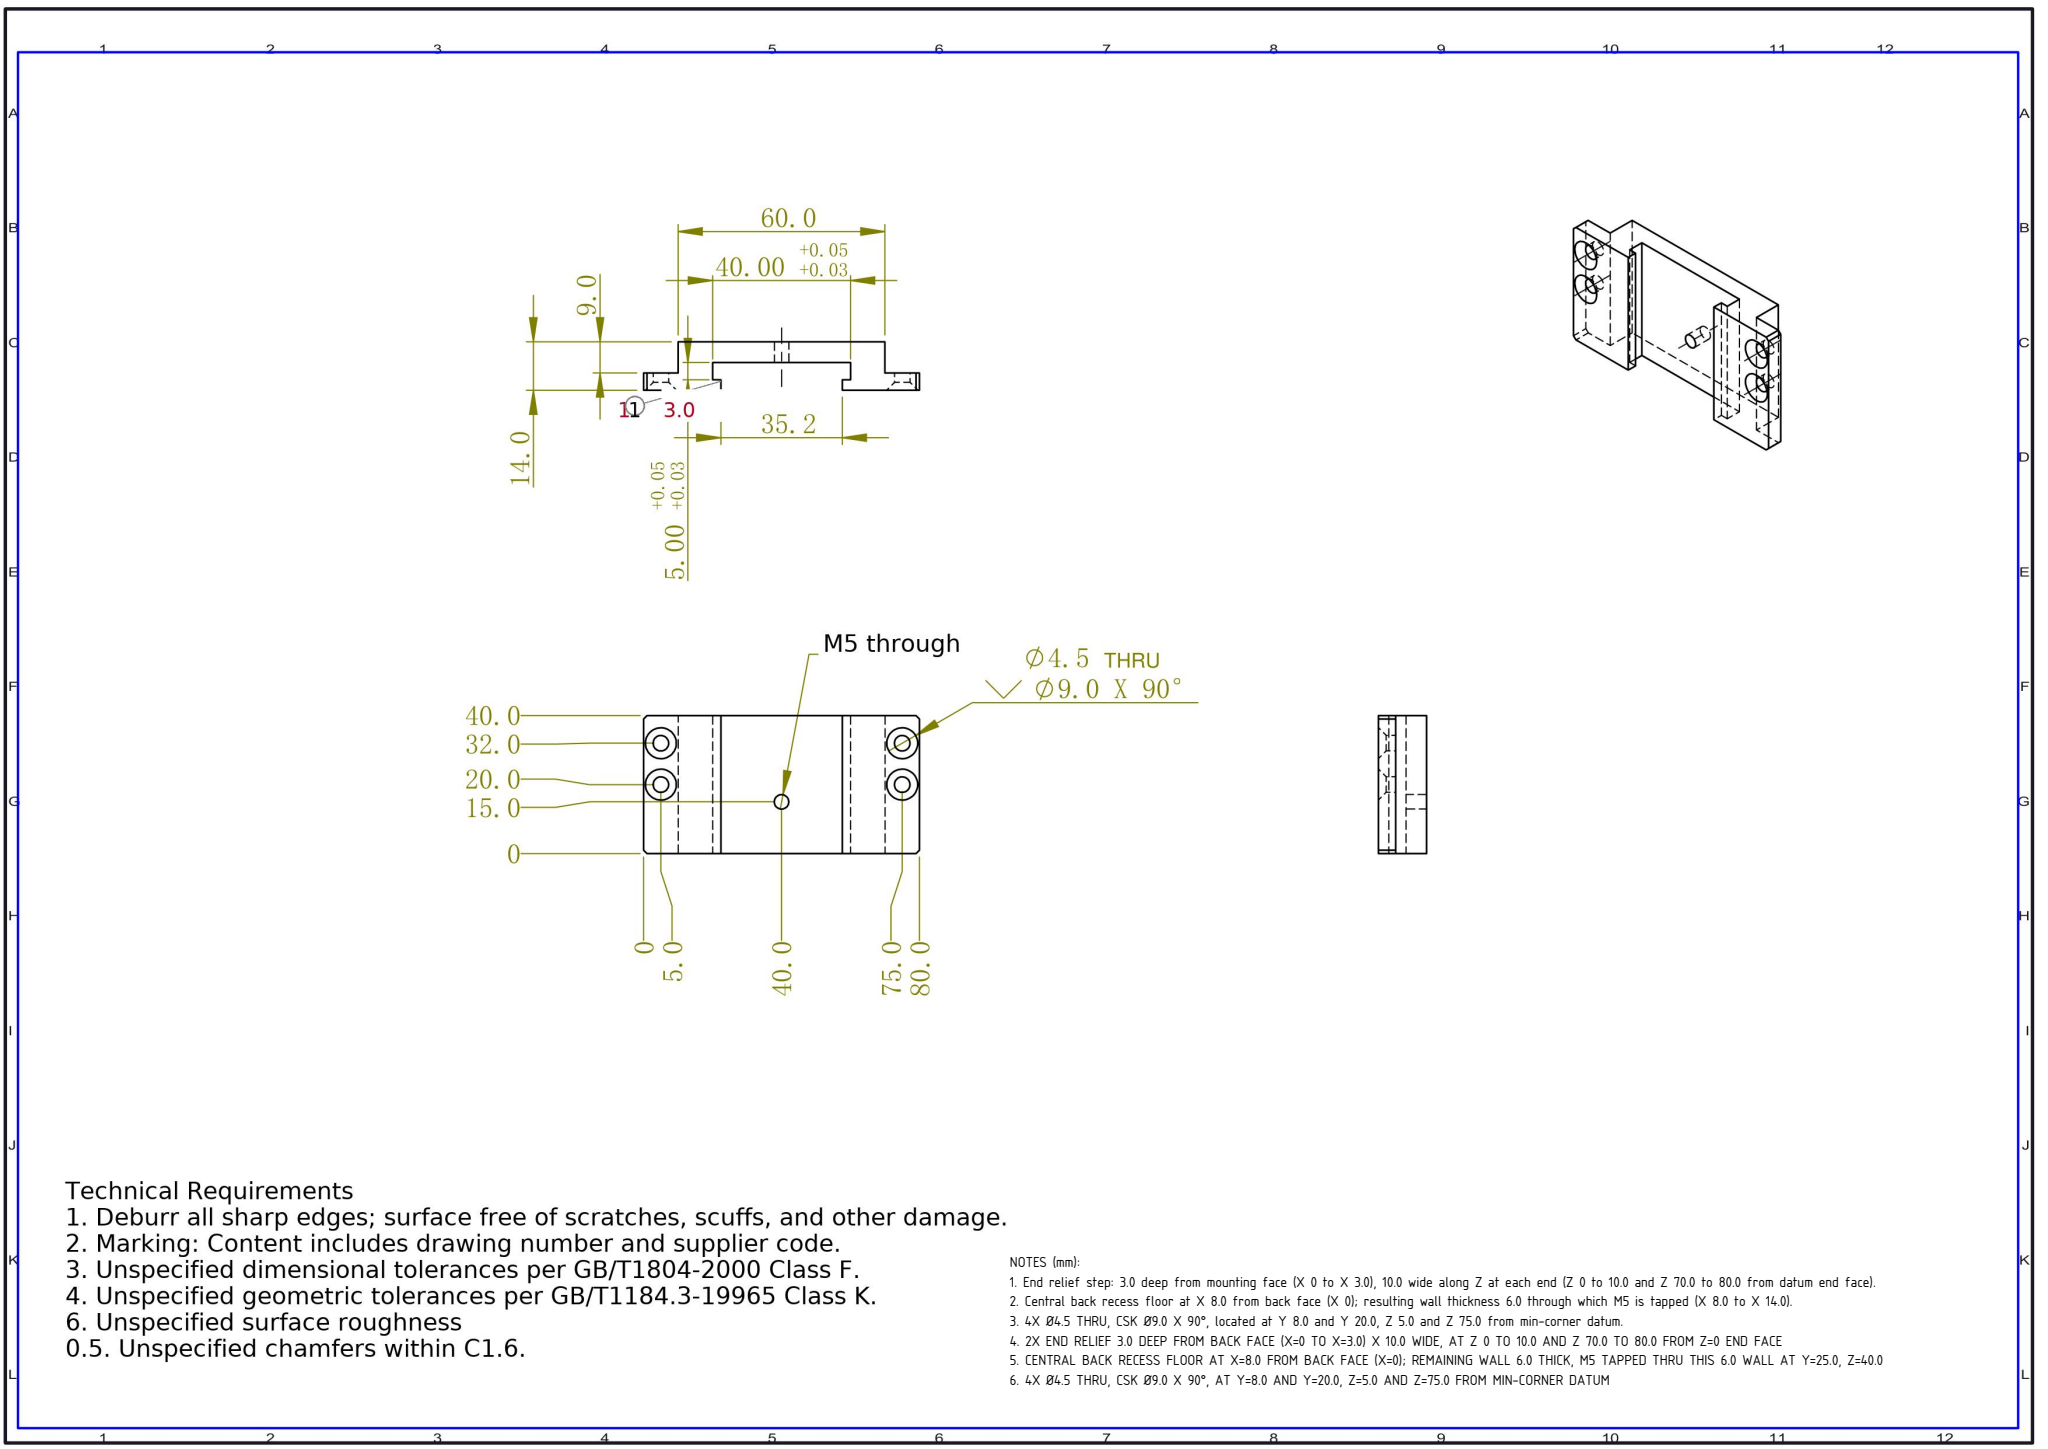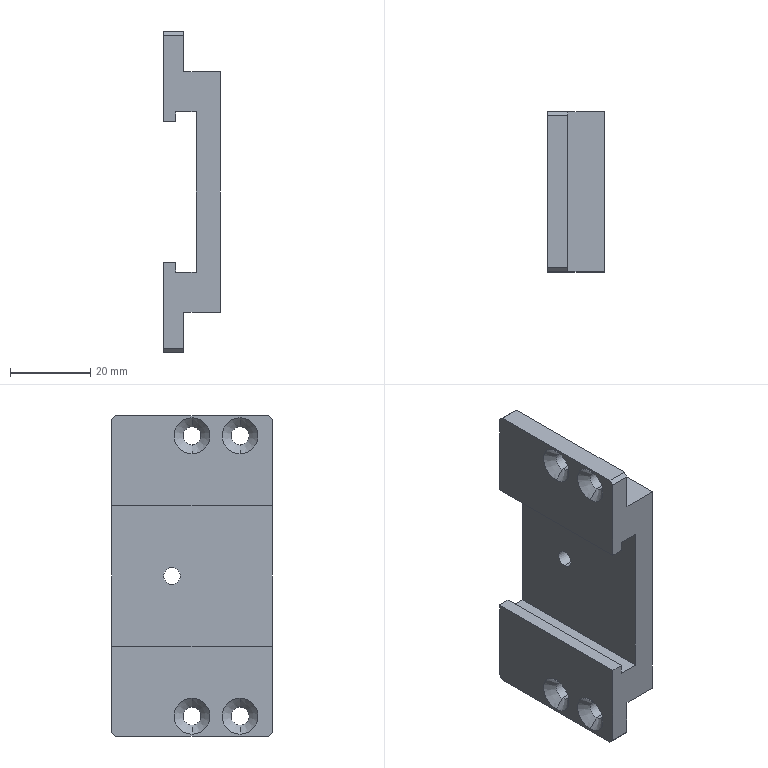Part | SolidWorks | mm | 1 solid | 40 faces | box 14 x 40 x 80 mm | volume 24778 mm3 | plane 22 | cylinder 10 | cone 8 | commonest cylinder face diameters 4.5 x8 4.2 x2
Drawing notes:
End relief step: 3.0 deep from mounting face (X 0 to X 3.0), 10.0 wide along Z at each end (Z 0 to 10.0 and Z 70.0 to 80.0 from datum end face). | from the solid: axis_planes x=3.0 with z=10.0 and z=70.0; bbox_xyz Z=80.0
Central back recess floor at X 8.0 from back face (X 0); resulting wall thickness 6.0 through which M5 is tapped (X 8.0 to X 14.0). | from the solid: axis_planes x=8.0 and x=14.0; cylinder dia 4.2 axis x length 6.0
4X Ø4.5 THRU, CSK Ø9.0 X 90°, located at Y 8.0 and Y 20.0, Z 5.0 and Z 75.0 from min-corner datum. | from the solid: cylinders dia 4.5 at (y=8.0,z=5.0),(y=8.0,z=75.0),(y=20.0,z=5.0),(y=20.0,z=75.0); cones 90.0 included angle ref_dia 8.96
2X END RELIEF 3.0 DEEP FROM BACK FACE (X=0 TO X=3.0) X 10.0 WIDE, AT Z 0 TO 10.0 AND Z 70.0 TO 80.0 FROM Z=0 END FACE | from the solid: axis_planes x=3.0 (count 2) with z=10.0 and z=70.0 planes; bbox_xyz Z=80.0
CENTRAL BACK RECESS FLOOR AT X=8.0 FROM BACK FACE (X=0); REMAINING WALL 6.0 THICK, M5 TAPPED THRU THIS 6.0 WALL AT Y=25.0, Z=40.0 | from the solid: axis_planes x=8.0 and x=14.0; cylinder dia 4.2 axis x at (y=25.0, z=40.0) length 6.0
4X Ø4.5 THRU, CSK Ø9.0 X 90°, AT Y=8.0 AND Y=20.0, Z=5.0 AND Z=75.0 FROM MIN-CORNER DATUM | from the solid: cylinders dia 4.5 axis x at (8,5),(8,75),(20,5),(20,75); cones 90.0 included angle ref_dia 8.96